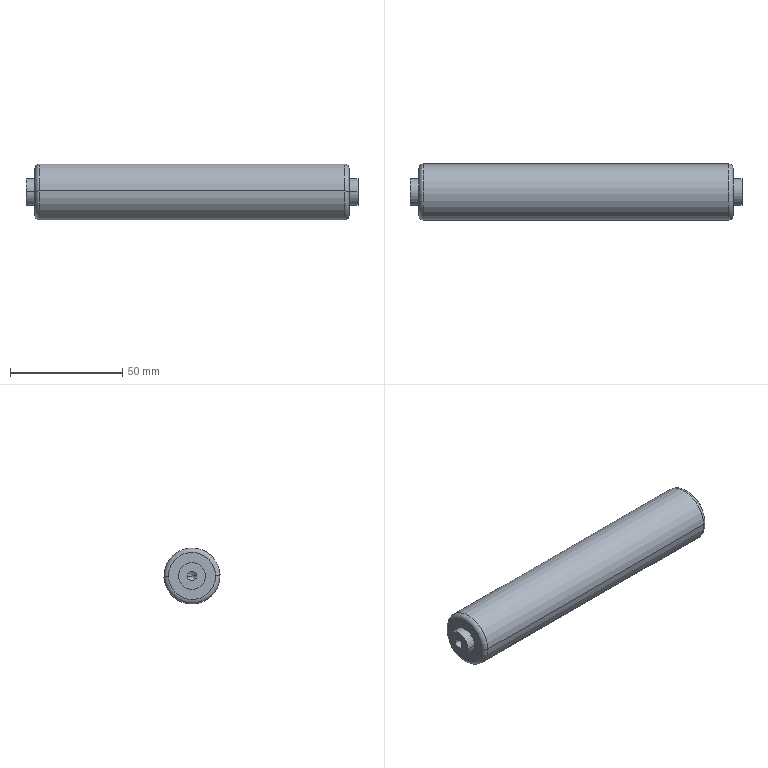Component | SolidWorks | GuideMechanism-1_StainlessSteelRoller-2 | 1 solid | 22 faces | box 148 x 25 x 25 mm | volume 69142 mm3 | cylinder 10 | cone 4 | torus 4 | plane 4 | commonest cylinder face diameters 4.2 x4 12 x4 25 x2
build123d program:
from build123d import *

# Parameters (mm, degrees)
FILLET1_R             = 2
SKETCH2_R             = 6
SKETCH2_R_2           = 4
BOSS_EXTRUDE1_DEPTH   = 4
BOSS_EXTRUDE2_START   = 4
SKETCH3_R             = 6
SKETCH3_R_2           = 4
BOSS_EXTRUDE2_DEPTH   = 4
M5_TAPPED_HOLE1_D     = 4.2
M5_TAPPED_HOLE1_DEPTH = 12.4
M5_TAPPED_HOLE1_TIP   = 1.262
M5_TAPPED_HOLE2_D     = 4.2
M5_TAPPED_HOLE2_DEPTH = 12.4
M5_TAPPED_HOLE2_TIP   = 1.262


with BuildPart() as part:
    # Sketch1 → Revolve1 (revolve)
    with BuildSketch(Plane(origin=(0, 0, 0), x_dir=(1, 0, 0), z_dir=(0, 1, 0)), mode=Mode.PRIVATE) as revolve1_sk:
        Polygon((0, 0), (0, 4), (4, 4), (4, 12.5), (144, 12.5), (144, 4), (148, 4), (148, 0), align=None)
    revolve(revolve1_sk.sketch.rotate(Axis((-146.184, 0, 0), (1, 0, 0)), 180), axis=Axis((-146.184, 0, 0), (1, 0, 0)))

    # Fillet1
    fillet1_edges = [part.edges().sort_by_distance(p)[0] for p in [
        (144, 0, -12.5),
        (4, 0, -12.5),
    ]]
    fillet(fillet1_edges, radius=FILLET1_R)

    # Sketch2 → Boss-Extrude1 (add)
    with BuildSketch(Plane.ZY.offset(-4)):
        with Locations(Location((0, 0, 0), (0, 0, 180))):
            Circle(SKETCH2_R)
        Circle(SKETCH2_R_2, mode=Mode.SUBTRACT)
    extrude(amount=BOSS_EXTRUDE1_DEPTH)

    # Sketch3 → Boss-Extrude2 (add)
    with BuildSketch(Plane(origin=(144, 0, 0), x_dir=(0, 0, -1), z_dir=(1, 0, 0)).offset(BOSS_EXTRUDE2_START)):
        Circle(SKETCH3_R)
        Circle(SKETCH3_R_2, mode=Mode.SUBTRACT)
    extrude(amount=-BOSS_EXTRUDE2_DEPTH)

    # M5 Tapped Hole1
    with Locations(Plane(origin=(148, 0, 0), x_dir=(0, 0, -1), z_dir=(1, 0, 0))):
        with Locations((0, 0)):
            Hole(M5_TAPPED_HOLE1_D / 2, depth=M5_TAPPED_HOLE1_DEPTH)
            with Locations((0, 0, -(M5_TAPPED_HOLE1_DEPTH + M5_TAPPED_HOLE1_TIP / 2))):  # 118° drill point
                Cone(0, M5_TAPPED_HOLE1_D / 2, M5_TAPPED_HOLE1_TIP, mode=Mode.SUBTRACT)

    # M5 Tapped Hole2
    with Locations(Plane(origin=(0, 0.1987, -0.07552), x_dir=(0, 0, 1), z_dir=(-1, 0, 0))):
        with Locations((0.07552, -0.1987)):
            Hole(M5_TAPPED_HOLE2_D / 2, depth=M5_TAPPED_HOLE2_DEPTH)
            with Locations((0, 0, -(M5_TAPPED_HOLE2_DEPTH + M5_TAPPED_HOLE2_TIP / 2))):  # 118° drill point
                Cone(0, M5_TAPPED_HOLE2_D / 2, M5_TAPPED_HOLE2_TIP, mode=Mode.SUBTRACT)


solid = part.part

# Placed as in the assembly
solid = solid.moved(Location((-513.272, -489.173, 1371.199), (0, 0, 0)))
STEP:
#1=COLOUR_RGB('',0.7922,0.8196,0.9333);
#2=FILL_AREA_STYLE_COLOUR('',#1);
#3=FILL_AREA_STYLE('',(#2));
#4=SURFACE_STYLE_FILL_AREA(#3);
#5=SURFACE_SIDE_STYLE('',(#4));
#6=SURFACE_STYLE_USAGE(.BOTH.,#5);
#7=PRESENTATION_STYLE_ASSIGNMENT((#6));
#8=CARTESIAN_POINT('',(-19.719,-19.176,53.981));
#9=VERTEX_POINT('',#8);
#10=CARTESIAN_POINT('',(-19.719,-19.341,53.987));
#11=VERTEX_POINT('',#10);
#12=CARTESIAN_POINT('',(-19.719,-19.259,53.984));
#13=DIRECTION('',(-1.,0.,0.));
#14=DIRECTION('',(0.,-0.9994,0.03596));
#15=AXIS2_PLACEMENT_3D('',#12,#13,#14);
#16=CIRCLE('',#15,0.08268);
#17=EDGE_CURVE('',#9,#11,#16,.T.);
#18=ORIENTED_EDGE('',*,*,#17,.F.);
#19=CARTESIAN_POINT('',(-20.208,-19.176,53.981));
#20=VERTEX_POINT('',#19);
#21=CARTESIAN_POINT('',(-20.208,-19.176,53.981));
#22=DIRECTION('',(-1.,0.,0.));
#23=VECTOR('',#22,39.37);
#24=LINE('',#21,#23);
#25=EDGE_CURVE('',#9,#20,#24,.T.);
#26=ORIENTED_EDGE('',*,*,#25,.T.);
#27=CARTESIAN_POINT('',(-20.208,-19.341,53.987));
#28=VERTEX_POINT('',#27);
#29=CARTESIAN_POINT('',(-20.208,-19.259,53.984));
#30=DIRECTION('',(-1.,0.,0.));
#31=DIRECTION('',(0.,-0.9994,0.03596));
#32=AXIS2_PLACEMENT_3D('',#29,#30,#31);
#33=CIRCLE('',#32,0.08268);
#34=EDGE_CURVE('',#20,#28,#33,.T.);
#35=ORIENTED_EDGE('',*,*,#34,.T.);
#36=CARTESIAN_POINT('',(-20.208,-19.341,53.987));
#37=DIRECTION('',(-1.,0.,0.));
#38=VECTOR('',#37,39.37);
#39=LINE('',#36,#38);
#40=EDGE_CURVE('',#11,#28,#39,.T.);
#41=ORIENTED_EDGE('',*,*,#40,.F.);
#42=EDGE_LOOP('',(#18,#26,#35,#41));
#43=FACE_OUTER_BOUND('',#42,.T.);
#44=CARTESIAN_POINT('',(-20.208,-19.259,53.984));
#45=DIRECTION('',(-1.,0.,0.));
#46=DIRECTION('',(0.,-0.9994,0.03596));
#47=AXIS2_PLACEMENT_3D('',#44,#45,#46);
#48=CYLINDRICAL_SURFACE('',#47,0.08268);
#49=ADVANCED_FACE('',(#43),#48,.F.);
#50=CARTESIAN_POINT('',(-19.67,-19.259,53.984));
#51=VERTEX_POINT('',#50);
#52=CARTESIAN_POINT('',(-19.719,-19.341,53.987));
#53=DIRECTION('',(-0.515,-0.8566,0.03082));
#54=VECTOR('',#53,39.37);
#55=LINE('',#52,#54);
#56=EDGE_CURVE('',#51,#11,#55,.T.);
#57=ORIENTED_EDGE('',*,*,#56,.F.);
#58=CARTESIAN_POINT('',(-19.719,-19.176,53.981));
#59=DIRECTION('',(-0.515,0.8566,-0.03082));
#60=VECTOR('',#59,39.37);
#61=LINE('',#58,#60);
#62=EDGE_CURVE('',#51,#9,#61,.T.);
#63=ORIENTED_EDGE('',*,*,#62,.T.);
#64=ORIENTED_EDGE('',*,*,#17,.T.);
#65=EDGE_LOOP('',(#57,#63,#64));
#66=FACE_OUTER_BOUND('',#65,.T.);
#67=CARTESIAN_POINT('',(-19.719,-19.259,53.984));
#68=DIRECTION('',(-1.,0.,0.));
#69=DIRECTION('',(0.,-0.9994,0.03596));
#70=AXIS2_PLACEMENT_3D('',#67,#68,#69);
#71=CONICAL_SURFACE('',#70,0.08268,1.03);
#72=ADVANCED_FACE('',(#66),#71,.F.);
#73=CARTESIAN_POINT('',(-14.869,-19.341,53.987));
#74=VERTEX_POINT('',#73);
#75=CARTESIAN_POINT('',(-14.869,-19.176,53.981));
#76=VERTEX_POINT('',#75);
#77=CARTESIAN_POINT('',(-14.869,-19.259,53.984));
#78=DIRECTION('',(1.,0.,0.));
#79=DIRECTION('',(0.,0.9994,-0.03596));
#80=AXIS2_PLACEMENT_3D('',#77,#78,#79);
#81=CIRCLE('',#80,0.08268);
#82=EDGE_CURVE('',#74,#76,#81,.T.);
#83=ORIENTED_EDGE('',*,*,#82,.F.);
#84=CARTESIAN_POINT('',(-14.381,-19.341,53.987));
#85=VERTEX_POINT('',#84);
#86=CARTESIAN_POINT('',(-14.381,-19.341,53.987));
#87=DIRECTION('',(1.,0.,0.));
#88=VECTOR('',#87,39.37);
#89=LINE('',#86,#88);
#90=EDGE_CURVE('',#74,#85,#89,.T.);
#91=ORIENTED_EDGE('',*,*,#90,.T.);
#92=CARTESIAN_POINT('',(-14.381,-19.176,53.981));
#93=VERTEX_POINT('',#92);
#94=CARTESIAN_POINT('',(-14.381,-19.259,53.984));
#95=DIRECTION('',(1.,0.,0.));
#96=DIRECTION('',(0.,0.9994,-0.03596));
#97=AXIS2_PLACEMENT_3D('',#94,#95,#96);
#98=CIRCLE('',#97,0.08268);
#99=EDGE_CURVE('',#85,#93,#98,.T.);
#100=ORIENTED_EDGE('',*,*,#99,.T.);
#101=CARTESIAN_POINT('',(-14.381,-19.176,53.981));
#102=DIRECTION('',(1.,0.,0.));
#103=VECTOR('',#102,39.37);
#104=LINE('',#101,#103);
#105=EDGE_CURVE('',#76,#93,#104,.T.);
#106=ORIENTED_EDGE('',*,*,#105,.F.);
#107=EDGE_LOOP('',(#83,#91,#100,#106));
#108=FACE_OUTER_BOUND('',#107,.T.);
#109=CARTESIAN_POINT('',(-14.381,-19.259,53.984));
#110=DIRECTION('',(1.,0.,0.));
#111=DIRECTION('',(0.,0.9994,-0.03596));
#112=AXIS2_PLACEMENT_3D('',#109,#110,#111);
#113=CYLINDRICAL_SURFACE('',#112,0.08268);
#114=ADVANCED_FACE('',(#108),#113,.F.);
#115=CARTESIAN_POINT('',(-14.919,-19.259,53.984));
#116=VERTEX_POINT('',#115);
#117=CARTESIAN_POINT('',(-14.869,-19.176,53.981));
#118=DIRECTION('',(0.515,0.8566,-0.03082));
#119=VECTOR('',#118,39.37);
#120=LINE('',#117,#119);
#121=EDGE_CURVE('',#116,#76,#120,.T.);
#122=ORIENTED_EDGE('',*,*,#121,.F.);
#123=CARTESIAN_POINT('',(-14.869,-19.341,53.987));
#124=DIRECTION('',(0.515,-0.8566,0.03082));
#125=VECTOR('',#124,39.37);
#126=LINE('',#123,#125);
#127=EDGE_CURVE('',#116,#74,#126,.T.);
#128=ORIENTED_EDGE('',*,*,#127,.T.);
#129=ORIENTED_EDGE('',*,*,#82,.T.);
#130=EDGE_LOOP('',(#122,#128,#129));
#131=FACE_OUTER_BOUND('',#130,.T.);
#132=CARTESIAN_POINT('',(-14.869,-19.259,53.984));
#133=DIRECTION('',(1.,0.,0.));
#134=DIRECTION('',(0.,0.9994,-0.03596));
#135=AXIS2_PLACEMENT_3D('',#132,#133,#134);
#136=CONICAL_SURFACE('',#135,0.08268,1.03);
#137=ADVANCED_FACE('',(#131),#136,.F.);
#138=CARTESIAN_POINT('',(-14.381,-19.023,53.976));
#139=VERTEX_POINT('',#138);
#140=CARTESIAN_POINT('',(-14.381,-19.495,53.993));
#141=VERTEX_POINT('',#140);
#142=CARTESIAN_POINT('',(-14.381,-19.259,53.984));
#143=DIRECTION('',(1.,0.,0.));
#144=DIRECTION('',(0.,0.9994,-0.03596));
#145=AXIS2_PLACEMENT_3D('',#142,#143,#144);
#146=CIRCLE('',#145,0.2362);
#147=EDGE_CURVE('',#139,#141,#146,.T.);
#148=ORIENTED_EDGE('',*,*,#147,.F.);
#149=CARTESIAN_POINT('',(-14.538,-19.023,53.976));
#150=VERTEX_POINT('',#149);
#151=CARTESIAN_POINT('',(-14.381,-19.023,53.976));
#152=DIRECTION('',(-1.,0.,0.));
#153=VECTOR('',#152,39.37);
#154=LINE('',#151,#153);
#155=EDGE_CURVE('',#139,#150,#154,.T.);
#156=ORIENTED_EDGE('',*,*,#155,.T.);
#157=CARTESIAN_POINT('',(-14.538,-19.495,53.993));
#158=VERTEX_POINT('',#157);
#159=CARTESIAN_POINT('',(-14.538,-19.259,53.984));
#160=DIRECTION('',(1.,0.,0.));
#161=DIRECTION('',(0.,-0.9994,0.03596));
#162=AXIS2_PLACEMENT_3D('',#159,#160,#161);
#163=CIRCLE('',#162,0.2362);
#164=EDGE_CURVE('',#150,#158,#163,.T.);
#165=ORIENTED_EDGE('',*,*,#164,.T.);
#166=CARTESIAN_POINT('',(-14.381,-19.495,53.993));
#167=DIRECTION('',(-1.,0.,0.));
#168=VECTOR('',#167,39.37);
#169=LINE('',#166,#168);
#170=EDGE_CURVE('',#141,#158,#169,.T.);
#171=ORIENTED_EDGE('',*,*,#170,.F.);
#172=EDGE_LOOP('',(#148,#156,#165,#171));
#173=FACE_OUTER_BOUND('',#172,.T.);
#174=CARTESIAN_POINT('',(-14.381,-19.259,53.984));
#175=DIRECTION('',(-1.,0.,0.));
#176=DIRECTION('',(0.,-0.9994,0.03596));
#177=AXIS2_PLACEMENT_3D('',#174,#175,#176);
#178=CYLINDRICAL_SURFACE('',#177,0.2362);
#179=ADVANCED_FACE('',(#173),#178,.T.);
#180=CARTESIAN_POINT('',(-20.208,-19.495,53.993));
#181=VERTEX_POINT('',#180);
#182=CARTESIAN_POINT('',(-20.208,-19.023,53.976));
#183=VERTEX_POINT('',#182);
#184=CARTESIAN_POINT('',(-20.208,-19.259,53.984));
#185=DIRECTION('',(-1.,0.,0.));
#186=DIRECTION('',(0.,-0.9994,0.03596));
#187=AXIS2_PLACEMENT_3D('',#184,#185,#186);
#188=CIRCLE('',#187,0.2362);
#189=EDGE_CURVE('',#181,#183,#188,.T.);
#190=ORIENTED_EDGE('',*,*,#189,.F.);
#191=CARTESIAN_POINT('',(-20.05,-19.495,53.993));
#192=VERTEX_POINT('',#191);
#193=CARTESIAN_POINT('',(-20.208,-19.495,53.993));
#194=DIRECTION('',(1.,0.,0.));
#195=VECTOR('',#194,39.37);
#196=LINE('',#193,#195);
#197=EDGE_CURVE('',#181,#192,#196,.T.);
#198=ORIENTED_EDGE('',*,*,#197,.T.);
#199=CARTESIAN_POINT('',(-20.05,-19.023,53.976));
#200=VERTEX_POINT('',#199);
#201=CARTESIAN_POINT('',(-20.05,-19.259,53.984));
#202=DIRECTION('',(-1.,0.,0.));
#203=DIRECTION('',(0.,0.9994,-0.03596));
#204=AXIS2_PLACEMENT_3D('',#201,#202,#203);
#205=CIRCLE('',#204,0.2362);
#206=EDGE_CURVE('',#192,#200,#205,.T.);
#207=ORIENTED_EDGE('',*,*,#206,.T.);
#208=CARTESIAN_POINT('',(-20.208,-19.023,53.976));
#209=DIRECTION('',(1.,0.,0.));
#210=VECTOR('',#209,39.37);
#211=LINE('',#208,#210);
#212=EDGE_CURVE('',#183,#200,#211,.T.);
#213=ORIENTED_EDGE('',*,*,#212,.F.);
#214=EDGE_LOOP('',(#190,#198,#207,#213));
#215=FACE_OUTER_BOUND('',#214,.T.);
#216=CARTESIAN_POINT('',(-20.208,-19.259,53.984));
#217=DIRECTION('',(1.,0.,0.));
#218=DIRECTION('',(0.,0.9994,-0.03596));
#219=AXIS2_PLACEMENT_3D('',#216,#217,#218);
#220=CYLINDRICAL_SURFACE('',#219,0.2362);
#221=ADVANCED_FACE('',(#215),#220,.T.);
#222=CARTESIAN_POINT('',(-20.05,-19.672,53.999));
#223=VERTEX_POINT('',#222);
#224=CARTESIAN_POINT('',(-20.05,-18.846,53.969));
#225=VERTEX_POINT('',#224);
#226=CARTESIAN_POINT('',(-20.05,-19.259,53.984));
#227=DIRECTION('',(-1.,0.,0.));
#228=DIRECTION('',(0.,0.9994,-0.03596));
#229=AXIS2_PLACEMENT_3D('',#226,#227,#228);
#230=CIRCLE('',#229,0.4134);
#231=EDGE_CURVE('',#223,#225,#230,.T.);
#232=ORIENTED_EDGE('',*,*,#231,.F.);
#233=CARTESIAN_POINT('',(-19.971,-19.751,54.002));
#234=VERTEX_POINT('',#233);
#235=CARTESIAN_POINT('',(-19.971,-19.672,53.999));
#236=DIRECTION('',(0.,0.03596,0.9994));
#237=DIRECTION('',(0.,-0.9994,0.03596));
#238=AXIS2_PLACEMENT_3D('',#235,#236,#237);
#239=CIRCLE('',#238,0.07874);
#240=EDGE_CURVE('',#223,#234,#239,.T.);
#241=ORIENTED_EDGE('',*,*,#240,.T.);
#242=CARTESIAN_POINT('',(-19.971,-18.767,53.966));
#243=VERTEX_POINT('',#242);
#244=CARTESIAN_POINT('',(-19.971,-19.259,53.984));
#245=DIRECTION('',(1.,0.,0.));
#246=DIRECTION('',(0.,0.9994,-0.03596));
#247=AXIS2_PLACEMENT_3D('',#244,#245,#246);
#248=CIRCLE('',#247,0.4921);
#249=EDGE_CURVE('',#243,#234,#248,.T.);
#250=ORIENTED_EDGE('',*,*,#249,.F.);
#251=CARTESIAN_POINT('',(-19.971,-18.846,53.969));
#252=DIRECTION('',(0.,-0.03596,-0.9994));
#253=DIRECTION('',(0.,0.9994,-0.03596));
#254=AXIS2_PLACEMENT_3D('',#251,#252,#253);
#255=CIRCLE('',#254,0.07874);
#256=EDGE_CURVE('',#225,#243,#255,.T.);
#257=ORIENTED_EDGE('',*,*,#256,.F.);
#258=EDGE_LOOP('',(#232,#241,#250,#257));
#259=FACE_OUTER_BOUND('',#258,.T.);
#260=CARTESIAN_POINT('',(-19.971,-19.259,53.984));
#261=DIRECTION('',(1.,0.,0.));
#262=DIRECTION('',(0.,0.9994,-0.03596));
#263=AXIS2_PLACEMENT_3D('',#260,#261,#262);
#264=TOROIDAL_SURFACE('',#263,0.4134,0.07874);
#265=ADVANCED_FACE('',(#259),#264,.T.);
#266=CARTESIAN_POINT('',(-14.538,-18.846,53.969));
#267=VERTEX_POINT('',#266);
#268=CARTESIAN_POINT('',(-14.538,-19.672,53.999));
#269=VERTEX_POINT('',#268);
#270=CARTESIAN_POINT('',(-14.538,-19.259,53.984));
#271=DIRECTION('',(1.,0.,0.));
#272=DIRECTION('',(0.,-0.9994,0.03596));
#273=AXIS2_PLACEMENT_3D('',#270,#271,#272);
#274=CIRCLE('',#273,0.4134);
#275=EDGE_CURVE('',#267,#269,#274,.T.);
#276=ORIENTED_EDGE('',*,*,#275,.F.);
#277=CARTESIAN_POINT('',(-14.617,-18.767,53.966));
#278=VERTEX_POINT('',#277);
#279=CARTESIAN_POINT('',(-14.617,-18.846,53.969));
#280=DIRECTION('',(0.,0.03596,0.9994));
#281=DIRECTION('',(0.,-0.9994,0.03596));
#282=AXIS2_PLACEMENT_3D('',#279,#280,#281);
#283=CIRCLE('',#282,0.07874);
#284=EDGE_CURVE('',#267,#278,#283,.T.);
#285=ORIENTED_EDGE('',*,*,#284,.T.);
#286=CARTESIAN_POINT('',(-14.617,-19.751,54.002));
#287=VERTEX_POINT('',#286);
#288=CARTESIAN_POINT('',(-14.617,-19.259,53.984));
#289=DIRECTION('',(-1.,0.,0.));
#290=DIRECTION('',(0.,-0.9994,0.03596));
#291=AXIS2_PLACEMENT_3D('',#288,#289,#290);
#292=CIRCLE('',#291,0.4921);
#293=EDGE_CURVE('',#287,#278,#292,.T.);
#294=ORIENTED_EDGE('',*,*,#293,.F.);
#295=CARTESIAN_POINT('',(-14.617,-19.672,53.999));
#296=DIRECTION('',(0.,-0.03596,-0.9994));
#297=DIRECTION('',(0.,0.9994,-0.03596));
#298=AXIS2_PLACEMENT_3D('',#295,#296,#297);
#299=CIRCLE('',#298,0.07874);
#300=EDGE_CURVE('',#269,#287,#299,.T.);
#301=ORIENTED_EDGE('',*,*,#300,.F.);
#302=EDGE_LOOP('',(#276,#285,#294,#301));
#303=FACE_OUTER_BOUND('',#302,.T.);
#304=CARTESIAN_POINT('',(-14.617,-19.259,53.984));
#305=DIRECTION('',(-1.,0.,0.));
#306=DIRECTION('',(0.,-0.9994,0.03596));
#307=AXIS2_PLACEMENT_3D('',#304,#305,#306);
#308=TOROIDAL_SURFACE('',#307,0.4134,0.07874);
#309=ADVANCED_FACE('',(#303),#308,.T.);
#310=ORIENTED_EDGE('',*,*,#293,.T.);
#311=CARTESIAN_POINT('',(-25.963,-18.767,53.966));
#312=DIRECTION('',(-1.,0.,0.));
#313=VECTOR('',#312,39.37);
#314=LINE('',#311,#313);
#315=EDGE_CURVE('',#278,#243,#314,.T.);
#316=ORIENTED_EDGE('',*,*,#315,.T.);
#317=ORIENTED_EDGE('',*,*,#249,.T.);
#318=CARTESIAN_POINT('',(-25.963,-19.751,54.002));
#319=DIRECTION('',(-1.,0.,0.));
#320=VECTOR('',#319,39.37);
#321=LINE('',#318,#320);
#322=EDGE_CURVE('',#287,#234,#321,.T.);
#323=ORIENTED_EDGE('',*,*,#322,.F.);
#324=EDGE_LOOP('',(#310,#316,#317,#323));
#325=FACE_OUTER_BOUND('',#324,.T.);
#326=CARTESIAN_POINT('',(-25.963,-19.259,53.984));
#327=DIRECTION('',(-1.,0.,0.));
#328=DIRECTION('',(0.,-0.9994,0.03596));
#329=AXIS2_PLACEMENT_3D('',#326,#327,#328);
#330=CYLINDRICAL_SURFACE('',#329,0.4921);
#331=ADVANCED_FACE('',(#325),#330,.T.);
#332=CARTESIAN_POINT('',(-14.538,-19.259,53.984));
#333=DIRECTION('',(1.,0.,0.));
#334=DIRECTION('',(0.,-0.9994,0.03596));
#335=AXIS2_PLACEMENT_3D('',#332,#333,#334);
#336=CIRCLE('',#335,0.4134);
#337=EDGE_CURVE('',#269,#267,#336,.T.);
#338=ORIENTED_EDGE('',*,*,#337,.T.);
#339=ORIENTED_EDGE('',*,*,#275,.T.);
#340=EDGE_LOOP('',(#338,#339));
#341=FACE_OUTER_BOUND('',#340,.T.);
#342=CARTESIAN_POINT('',(-14.538,-19.259,53.984));
#343=DIRECTION('',(1.,0.,0.));
#344=DIRECTION('',(0.,-0.9994,0.03596));
#345=AXIS2_PLACEMENT_3D('',#342,#343,#344);
#346=CIRCLE('',#345,0.2362);
#347=EDGE_CURVE('',#158,#150,#346,.T.);
#348=ORIENTED_EDGE('',*,*,#347,.F.);
#349=ORIENTED_EDGE('',*,*,#164,.F.);
#350=EDGE_LOOP('',(#348,#349));
#351=FACE_BOUND('',#350,.T.);
#352=CARTESIAN_POINT('',(-14.538,-18.767,53.966));
#353=DIRECTION('',(-1.,0.,0.));
#354=DIRECTION('',(0.,-0.9994,0.03596));
#355=AXIS2_PLACEMENT_3D('',#352,#353,#354);
#356=PLANE('',#355);
#357=ADVANCED_FACE('',(#341,#351),#356,.F.);
#358=CARTESIAN_POINT('',(-20.05,-19.259,53.984));
#359=DIRECTION('',(-1.,0.,0.));
#360=DIRECTION('',(0.,0.9994,-0.03596));
#361=AXIS2_PLACEMENT_3D('',#358,#359,#360);
#362=CIRCLE('',#361,0.4134);
#363=EDGE_CURVE('',#225,#223,#362,.T.);
#364=ORIENTED_EDGE('',*,*,#363,.T.);
#365=ORIENTED_EDGE('',*,*,#231,.T.);
#366=EDGE_LOOP('',(#364,#365));
#367=FACE_OUTER_BOUND('',#366,.T.);
#368=CARTESIAN_POINT('',(-20.05,-19.259,53.984));
#369=DIRECTION('',(-1.,0.,0.));
#370=DIRECTION('',(0.,0.9994,-0.03596));
#371=AXIS2_PLACEMENT_3D('',#368,#369,#370);
#372=CIRCLE('',#371,0.2362);
#373=EDGE_CURVE('',#200,#192,#372,.T.);
#374=ORIENTED_EDGE('',*,*,#373,.F.);
#375=ORIENTED_EDGE('',*,*,#206,.F.);
#376=EDGE_LOOP('',(#374,#375));
#377=FACE_BOUND('',#376,.T.);
#378=CARTESIAN_POINT('',(-20.05,-19.101,53.979));
#379=DIRECTION('',(1.,0.,0.));
#380=DIRECTION('',(0.,0.9994,-0.03596));
#381=AXIS2_PLACEMENT_3D('',#378,#379,#380);
#382=PLANE('',#381);
#383=ADVANCED_FACE('',(#367,#377),#382,.F.);
#384=ORIENTED_EDGE('',*,*,#315,.F.);
#385=CARTESIAN_POINT('',(-14.617,-19.259,53.984));
#386=DIRECTION('',(-1.,0.,0.));
#387=DIRECTION('',(0.,-0.9994,0.03596));
#388=AXIS2_PLACEMENT_3D('',#385,#386,#387);
#389=CIRCLE('',#388,0.4921);
#390=EDGE_CURVE('',#278,#287,#389,.T.);
#391=ORIENTED_EDGE('',*,*,#390,.T.);
#392=ORIENTED_EDGE('',*,*,#322,.T.);
#393=CARTESIAN_POINT('',(-19.971,-19.259,53.984));
#394=DIRECTION('',(1.,0.,0.));
#395=DIRECTION('',(0.,0.9994,-0.03596));
#396=AXIS2_PLACEMENT_3D('',#393,#394,#395);
#397=CIRCLE('',#396,0.4921);
#398=EDGE_CURVE('',#234,#243,#397,.T.);
#399=ORIENTED_EDGE('',*,*,#398,.T.);
#400=EDGE_LOOP('',(#384,#391,#392,#399));
#401=FACE_OUTER_BOUND('',#400,.T.);
#402=CARTESIAN_POINT('',(-25.963,-19.259,53.984));
#403=DIRECTION('',(-1.,0.,0.));
#404=DIRECTION('',(0.,-0.9994,0.03596));
#405=AXIS2_PLACEMENT_3D('',#402,#403,#404);
#406=CYLINDRICAL_SURFACE('',#405,0.4921);
#407=ADVANCED_FACE('',(#401),#406,.T.);
#408=ORIENTED_EDGE('',*,*,#284,.F.);
#409=ORIENTED_EDGE('',*,*,#337,.F.);
#410=ORIENTED_EDGE('',*,*,#300,.T.);
#411=ORIENTED_EDGE('',*,*,#390,.F.);
#412=EDGE_LOOP('',(#408,#409,#410,#411));
#413=FACE_OUTER_BOUND('',#412,.T.);
#414=CARTESIAN_POINT('',(-14.617,-19.259,53.984));
#415=DIRECTION('',(-1.,0.,0.));
#416=DIRECTION('',(0.,-0.9994,0.03596));
#417=AXIS2_PLACEMENT_3D('',#414,#415,#416);
#418=TOROIDAL_SURFACE('',#417,0.4134,0.07874);
#419=ADVANCED_FACE('',(#413),#418,.T.);
#420=ORIENTED_EDGE('',*,*,#240,.F.);
#421=ORIENTED_EDGE('',*,*,#363,.F.);
#422=ORIENTED_EDGE('',*,*,#256,.T.);
#423=ORIENTED_EDGE('',*,*,#398,.F.);
#424=EDGE_LOOP('',(#420,#421,#422,#423));
#425=FACE_OUTER_BOUND('',#424,.T.);
#426=CARTESIAN_POINT('',(-19.971,-19.259,53.984));
#427=DIRECTION('',(1.,0.,0.));
#428=DIRECTION('',(0.,0.9994,-0.03596));
#429=AXIS2_PLACEMENT_3D('',#426,#427,#428);
#430=TOROIDAL_SURFACE('',#429,0.4134,0.07874);
#431=ADVANCED_FACE('',(#425),#430,.T.);
#432=ORIENTED_EDGE('',*,*,#197,.F.);
#433=CARTESIAN_POINT('',(-20.208,-19.259,53.984));
#434=DIRECTION('',(-1.,0.,0.));
#435=DIRECTION('',(0.,-0.9994,0.03596));
#436=AXIS2_PLACEMENT_3D('',#433,#434,#435);
#437=CIRCLE('',#436,0.2362);
#438=EDGE_CURVE('',#183,#181,#437,.T.);
#439=ORIENTED_EDGE('',*,*,#438,.F.);
#440=ORIENTED_EDGE('',*,*,#212,.T.);
#441=ORIENTED_EDGE('',*,*,#373,.T.);
#442=EDGE_LOOP('',(#432,#439,#440,#441));
#443=FACE_OUTER_BOUND('',#442,.T.);
#444=CARTESIAN_POINT('',(-20.208,-19.259,53.984));
#445=DIRECTION('',(1.,0.,0.));
#446=DIRECTION('',(0.,0.9994,-0.03596));
#447=AXIS2_PLACEMENT_3D('',#444,#445,#446);
#448=CYLINDRICAL_SURFACE('',#447,0.2362);
#449=ADVANCED_FACE('',(#443),#448,.T.);
#450=CARTESIAN_POINT('',(-20.208,-19.259,53.984));
#451=DIRECTION('',(-1.,0.,0.));
#452=DIRECTION('',(0.,-0.9994,0.03596));
#453=AXIS2_PLACEMENT_3D('',#450,#451,#452);
#454=CIRCLE('',#453,0.08268);
#455=EDGE_CURVE('',#28,#20,#454,.T.);
#456=ORIENTED_EDGE('',*,*,#455,.F.);
#457=ORIENTED_EDGE('',*,*,#34,.F.);
#458=EDGE_LOOP('',(#456,#457));
#459=FACE_BOUND('',#458,.T.);
#460=ORIENTED_EDGE('',*,*,#438,.T.);
#461=ORIENTED_EDGE('',*,*,#189,.T.);
#462=EDGE_LOOP('',(#460,#461));
#463=FACE_OUTER_BOUND('',#462,.T.);
#464=CARTESIAN_POINT('',(-20.208,-19.259,53.984));
#465=DIRECTION('',(1.,0.,0.));
#466=DIRECTION('',(0.,0.9994,-0.03596));
#467=AXIS2_PLACEMENT_3D('',#464,#465,#466);
#468=PLANE('',#467);
#469=ADVANCED_FACE('',(#459,#463),#468,.F.);
#470=ORIENTED_EDGE('',*,*,#155,.F.);
#471=CARTESIAN_POINT('',(-14.381,-19.259,53.984));
#472=DIRECTION('',(1.,0.,0.));
#473=DIRECTION('',(0.,0.9994,-0.03596));
#474=AXIS2_PLACEMENT_3D('',#471,#472,#473);
#475=CIRCLE('',#474,0.2362);
#476=EDGE_CURVE('',#141,#139,#475,.T.);
#477=ORIENTED_EDGE('',*,*,#476,.F.);
#478=ORIENTED_EDGE('',*,*,#170,.T.);
#479=ORIENTED_EDGE('',*,*,#347,.T.);
#480=EDGE_LOOP('',(#470,#477,#478,#479));
#481=FACE_OUTER_BOUND('',#480,.T.);
#482=CARTESIAN_POINT('',(-14.381,-19.259,53.984));
#483=DIRECTION('',(-1.,0.,0.));
#484=DIRECTION('',(0.,-0.9994,0.03596));
#485=AXIS2_PLACEMENT_3D('',#482,#483,#484);
#486=CYLINDRICAL_SURFACE('',#485,0.2362);
#487=ADVANCED_FACE('',(#481),#486,.T.);
#488=CARTESIAN_POINT('',(-14.381,-19.259,53.984));
#489=DIRECTION('',(1.,0.,0.));
#490=DIRECTION('',(0.,0.9994,-0.03596));
#491=AXIS2_PLACEMENT_3D('',#488,#489,#490);
#492=CIRCLE('',#491,0.08268);
#493=EDGE_CURVE('',#93,#85,#492,.T.);
#494=ORIENTED_EDGE('',*,*,#493,.F.);
#495=ORIENTED_EDGE('',*,*,#99,.F.);
#496=EDGE_LOOP('',(#494,#495));
#497=FACE_BOUND('',#496,.T.);
#498=ORIENTED_EDGE('',*,*,#476,.T.);
#499=ORIENTED_EDGE('',*,*,#147,.T.);
#500=EDGE_LOOP('',(#498,#499));
#501=FACE_OUTER_BOUND('',#500,.T.);
#502=CARTESIAN_POINT('',(-14.381,-19.101,53.979));
#503=DIRECTION('',(-1.,0.,0.));
#504=DIRECTION('',(0.,-0.9994,0.03596));
#505=AXIS2_PLACEMENT_3D('',#502,#503,#504);
#506=PLANE('',#505);
#507=ADVANCED_FACE('',(#497,#501),#506,.F.);
#508=ORIENTED_EDGE('',*,*,#127,.F.);
#509=ORIENTED_EDGE('',*,*,#121,.T.);
#510=CARTESIAN_POINT('',(-14.869,-19.259,53.984));
#511=DIRECTION('',(1.,0.,0.));
#512=DIRECTION('',(0.,0.9994,-0.03596));
#513=AXIS2_PLACEMENT_3D('',#510,#511,#512);
#514=CIRCLE('',#513,0.08268);
#515=EDGE_CURVE('',#76,#74,#514,.T.);
#516=ORIENTED_EDGE('',*,*,#515,.T.);
#517=EDGE_LOOP('',(#508,#509,#516));
#518=FACE_OUTER_BOUND('',#517,.T.);
#519=CARTESIAN_POINT('',(-14.869,-19.259,53.984));
#520=DIRECTION('',(1.,0.,0.));
#521=DIRECTION('',(0.,0.9994,-0.03596));
#522=AXIS2_PLACEMENT_3D('',#519,#520,#521);
#523=CONICAL_SURFACE('',#522,0.08268,1.03);
#524=ADVANCED_FACE('',(#518),#523,.F.);
#525=ORIENTED_EDGE('',*,*,#90,.F.);
#526=ORIENTED_EDGE('',*,*,#515,.F.);
#527=ORIENTED_EDGE('',*,*,#105,.T.);
#528=ORIENTED_EDGE('',*,*,#493,.T.);
#529=EDGE_LOOP('',(#525,#526,#527,#528));
#530=FACE_OUTER_BOUND('',#529,.T.);
#531=CARTESIAN_POINT('',(-14.381,-19.259,53.984));
#532=DIRECTION('',(1.,0.,0.));
#533=DIRECTION('',(0.,0.9994,-0.03596));
#534=AXIS2_PLACEMENT_3D('',#531,#532,#533);
#535=CYLINDRICAL_SURFACE('',#534,0.08268);
#536=ADVANCED_FACE('',(#530),#535,.F.);
#537=ORIENTED_EDGE('',*,*,#62,.F.);
#538=ORIENTED_EDGE('',*,*,#56,.T.);
#539=CARTESIAN_POINT('',(-19.719,-19.259,53.984));
#540=DIRECTION('',(-1.,0.,0.));
#541=DIRECTION('',(0.,-0.9994,0.03596));
#542=AXIS2_PLACEMENT_3D('',#539,#540,#541);
#543=CIRCLE('',#542,0.08268);
#544=EDGE_CURVE('',#11,#9,#543,.T.);
#545=ORIENTED_EDGE('',*,*,#544,.T.);
#546=EDGE_LOOP('',(#537,#538,#545));
#547=FACE_OUTER_BOUND('',#546,.T.);
#548=CARTESIAN_POINT('',(-19.719,-19.259,53.984));
#549=DIRECTION('',(-1.,0.,0.));
#550=DIRECTION('',(0.,-0.9994,0.03596));
#551=AXIS2_PLACEMENT_3D('',#548,#549,#550);
#552=CONICAL_SURFACE('',#551,0.08268,1.03);
#553=ADVANCED_FACE('',(#547),#552,.F.);
#554=ORIENTED_EDGE('',*,*,#25,.F.);
#555=ORIENTED_EDGE('',*,*,#544,.F.);
#556=ORIENTED_EDGE('',*,*,#40,.T.);
#557=ORIENTED_EDGE('',*,*,#455,.T.);
#558=EDGE_LOOP('',(#554,#555,#556,#557));
#559=FACE_OUTER_BOUND('',#558,.T.);
#560=CARTESIAN_POINT('',(-20.208,-19.259,53.984));
#561=DIRECTION('',(-1.,0.,0.));
#562=DIRECTION('',(0.,-0.9994,0.03596));
#563=AXIS2_PLACEMENT_3D('',#560,#561,#562);
#564=CYLINDRICAL_SURFACE('',#563,0.08268);
#565=ADVANCED_FACE('',(#559),#564,.F.);
#566=CLOSED_SHELL('',(#49,#72,#114,#137,#179,#221,#265,#309,#331,#357,#383,#407,#419,#431,#449,#469,#487,#507,#524,#536,#553,#565));
#567=MANIFOLD_SOLID_BREP('',#566);
#568=STYLED_ITEM('',(#7),#567);
#569=PRESENTATION_LAYER_ASSIGNMENT('','',(#568));
#570=(LENGTH_UNIT()NAMED_UNIT(*)SI_UNIT($,.METRE.));
#571=LENGTH_MEASURE_WITH_UNIT(LENGTH_MEASURE(0.0254),#570);
#572=DIMENSIONAL_EXPONENTS(1.,0.,0.,0.,0.,0.,0.);
#573=(CONVERSION_BASED_UNIT('',#571)LENGTH_UNIT()NAMED_UNIT(#572));
#574=UNCERTAINTY_MEASURE_WITH_UNIT(LENGTH_MEASURE(0.00001),#573,'','');
#575=(NAMED_UNIT(*)PLANE_ANGLE_UNIT()SI_UNIT($,.RADIAN.));
#576=(NAMED_UNIT(*)SI_UNIT($,.STERADIAN.)SOLID_ANGLE_UNIT());
#577=(GEOMETRIC_REPRESENTATION_CONTEXT(3)GLOBAL_UNCERTAINTY_ASSIGNED_CONTEXT((#574))GLOBAL_UNIT_ASSIGNED_CONTEXT((#573,#575,#576))REPRESENTATION_CONTEXT('',''));
#578=MECHANICAL_DESIGN_GEOMETRIC_PRESENTATION_REPRESENTATION('',(#568),#577);
#579=CARTESIAN_POINT('',(0.,0.,0.));
#580=DIRECTION('',(0.,0.,1.));
#581=DIRECTION('',(1.,0.,0.));
#582=AXIS2_PLACEMENT_3D('',#579,#580,#581);
#583=(LENGTH_UNIT()NAMED_UNIT(*)SI_UNIT($,.METRE.));
#584=LENGTH_MEASURE_WITH_UNIT(LENGTH_MEASURE(0.0254),#583);
#585=DIMENSIONAL_EXPONENTS(1.,0.,0.,0.,0.,0.,0.);
#586=(CONVERSION_BASED_UNIT('',#584)LENGTH_UNIT()NAMED_UNIT(#585));
#587=UNCERTAINTY_MEASURE_WITH_UNIT(LENGTH_MEASURE(0.00001),#586,'','');
#588=(NAMED_UNIT(*)PLANE_ANGLE_UNIT()SI_UNIT($,.RADIAN.));
#589=(NAMED_UNIT(*)SI_UNIT($,.STERADIAN.)SOLID_ANGLE_UNIT());
#590=(GEOMETRIC_REPRESENTATION_CONTEXT(3)GLOBAL_UNCERTAINTY_ASSIGNED_CONTEXT((#587))GLOBAL_UNIT_ASSIGNED_CONTEXT((#586,#588,#589))REPRESENTATION_CONTEXT('',''));
#591=ADVANCED_BREP_SHAPE_REPRESENTATION('',(#567,#582),#590);